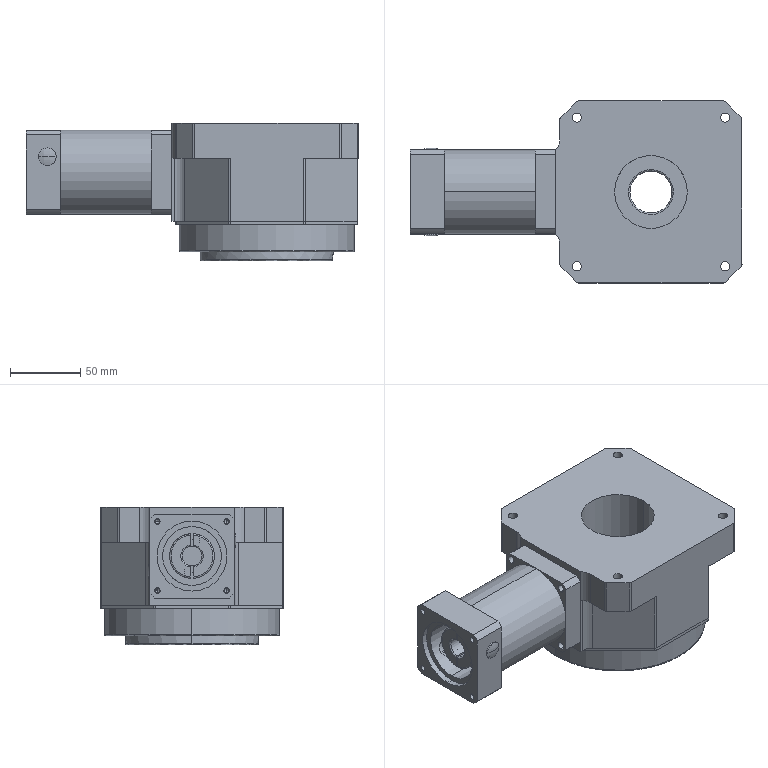Component | SolidWorks | V1ZHXTRR60SecondarySB1-1_V1ZHXT1,RR60BodySB1-1 | 3 solids | 414 faces | box 237 x 130 x 98.5 mm | volume 1476253 mm3 | cylinder 218 | plane 105 | cone 73 | spline 18 | commonest cylinder face diameters 3.4 x32 4 x30 5.02 x16 5.5 x16 5 x16 4.2 x16 3.3 x8 80 x8